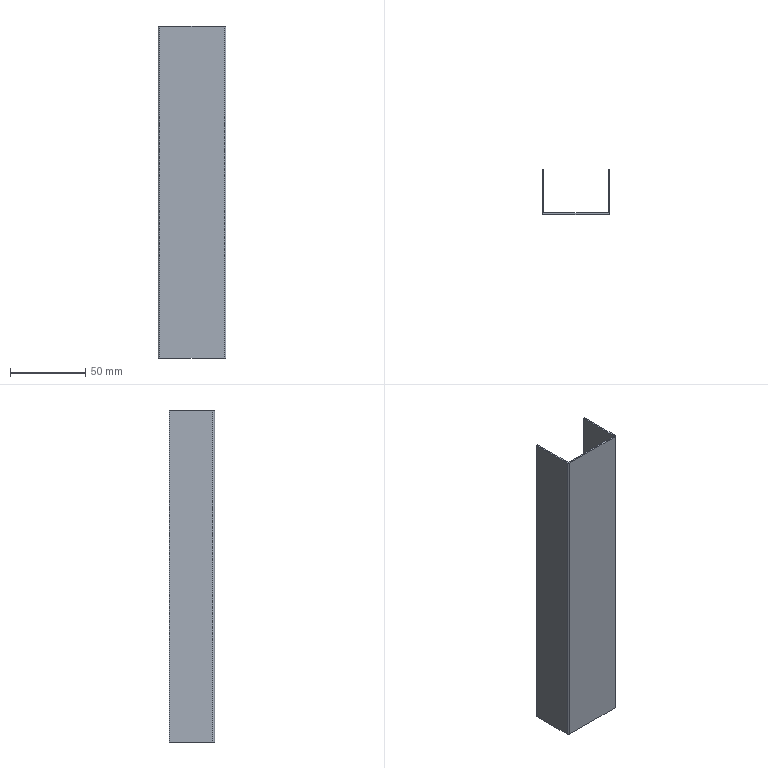Component | SolidWorks | WeldmentDrawing-1_WireDuct-1 | 1 solid | 22 faces | box 45 x 30 x 220 mm | volume 22547 mm3 | plane 18 | cylinder 4 | commonest cylinder face diameters 2.2 x2 0.2 x2
STEP:
#1=COLOUR_RGB('',0.7922,0.8196,0.9333);
#2=FILL_AREA_STYLE_COLOUR('',#1);
#3=FILL_AREA_STYLE('',(#2));
#4=SURFACE_STYLE_FILL_AREA(#3);
#5=SURFACE_SIDE_STYLE('',(#4));
#6=SURFACE_STYLE_USAGE(.BOTH.,#5);
#7=PRESENTATION_STYLE_ASSIGNMENT((#6));
#8=CARTESIAN_POINT('',(-6.554,2.411,-7.874));
#9=VERTEX_POINT('',#8);
#10=CARTESIAN_POINT('',(-8.239,2.411,-7.874));
#11=VERTEX_POINT('',#10);
#12=CARTESIAN_POINT('',(-8.282,2.411,-7.874));
#13=DIRECTION('',(-1.,0.,0.));
#14=VECTOR('',#13,39.37);
#15=LINE('',#12,#14);
#16=EDGE_CURVE('',#9,#11,#15,.T.);
#17=ORIENTED_EDGE('',*,*,#16,.F.);
#18=CARTESIAN_POINT('',(-6.554,2.411,0.7874));
#19=VERTEX_POINT('',#18);
#20=CARTESIAN_POINT('',(-6.554,2.411,-7.874));
#21=DIRECTION('',(0.,0.,1.));
#22=VECTOR('',#21,39.37);
#23=LINE('',#20,#22);
#24=EDGE_CURVE('',#9,#19,#23,.T.);
#25=ORIENTED_EDGE('',*,*,#24,.T.);
#26=CARTESIAN_POINT('',(-8.239,2.411,0.7874));
#27=VERTEX_POINT('',#26);
#28=CARTESIAN_POINT('',(-8.282,2.411,0.7874));
#29=DIRECTION('',(1.,0.,0.));
#30=VECTOR('',#29,39.37);
#31=LINE('',#28,#30);
#32=EDGE_CURVE('',#27,#19,#31,.T.);
#33=ORIENTED_EDGE('',*,*,#32,.F.);
#34=CARTESIAN_POINT('',(-8.239,2.411,0.7874));
#35=DIRECTION('',(0.,0.,-1.));
#36=VECTOR('',#35,39.37);
#37=LINE('',#34,#36);
#38=EDGE_CURVE('',#27,#11,#37,.T.);
#39=ORIENTED_EDGE('',*,*,#38,.T.);
#40=EDGE_LOOP('',(#17,#25,#33,#39));
#41=FACE_OUTER_BOUND('',#40,.T.);
#42=CARTESIAN_POINT('',(-6.765,2.411,-1.381));
#43=DIRECTION('',(0.,-1.,0.));
#44=DIRECTION('',(0.,0.,-1.));
#45=AXIS2_PLACEMENT_3D('',#42,#43,#44);
#46=PLANE('',#45);
#47=ADVANCED_FACE('',(#41),#46,.T.);
#48=CARTESIAN_POINT('',(-6.554,2.451,-7.874));
#49=VERTEX_POINT('',#48);
#50=CARTESIAN_POINT('',(-6.554,2.451,0.7874));
#51=VERTEX_POINT('',#50);
#52=CARTESIAN_POINT('',(-6.554,2.451,-7.874));
#53=DIRECTION('',(0.,0.,1.));
#54=VECTOR('',#53,39.37);
#55=LINE('',#52,#54);
#56=EDGE_CURVE('',#49,#51,#55,.T.);
#57=ORIENTED_EDGE('',*,*,#56,.F.);
#58=CARTESIAN_POINT('',(-8.239,2.451,-7.874));
#59=VERTEX_POINT('',#58);
#60=CARTESIAN_POINT('',(-8.282,2.451,-7.874));
#61=DIRECTION('',(-1.,0.,0.));
#62=VECTOR('',#61,39.37);
#63=LINE('',#60,#62);
#64=EDGE_CURVE('',#49,#59,#63,.T.);
#65=ORIENTED_EDGE('',*,*,#64,.T.);
#66=CARTESIAN_POINT('',(-8.239,2.451,0.7874));
#67=VERTEX_POINT('',#66);
#68=CARTESIAN_POINT('',(-8.239,2.451,0.7874));
#69=DIRECTION('',(0.,0.,-1.));
#70=VECTOR('',#69,39.37);
#71=LINE('',#68,#70);
#72=EDGE_CURVE('',#67,#59,#71,.T.);
#73=ORIENTED_EDGE('',*,*,#72,.F.);
#74=CARTESIAN_POINT('',(-8.282,2.451,0.7874));
#75=DIRECTION('',(1.,0.,0.));
#76=VECTOR('',#75,39.37);
#77=LINE('',#74,#76);
#78=EDGE_CURVE('',#67,#51,#77,.T.);
#79=ORIENTED_EDGE('',*,*,#78,.T.);
#80=EDGE_LOOP('',(#57,#65,#73,#79));
#81=FACE_OUTER_BOUND('',#80,.T.);
#82=CARTESIAN_POINT('',(-6.765,2.451,-1.381));
#83=DIRECTION('',(0.,-1.,0.));
#84=DIRECTION('',(0.,0.,-1.));
#85=AXIS2_PLACEMENT_3D('',#82,#83,#84);
#86=PLANE('',#85);
#87=ADVANCED_FACE('',(#81),#86,.F.);
#88=ORIENTED_EDGE('',*,*,#64,.F.);
#89=CARTESIAN_POINT('',(-6.554,2.451,-7.874));
#90=DIRECTION('',(0.,-1.,0.));
#91=VECTOR('',#90,39.37);
#92=LINE('',#89,#91);
#93=EDGE_CURVE('',#49,#9,#92,.T.);
#94=ORIENTED_EDGE('',*,*,#93,.T.);
#95=ORIENTED_EDGE('',*,*,#16,.T.);
#96=CARTESIAN_POINT('',(-8.239,2.451,-7.874));
#97=DIRECTION('',(0.,-1.,0.));
#98=VECTOR('',#97,39.37);
#99=LINE('',#96,#98);
#100=EDGE_CURVE('',#59,#11,#99,.T.);
#101=ORIENTED_EDGE('',*,*,#100,.F.);
#102=EDGE_LOOP('',(#88,#94,#95,#101));
#103=FACE_OUTER_BOUND('',#102,.T.);
#104=CARTESIAN_POINT('',(-8.282,2.411,-7.874));
#105=DIRECTION('',(0.,0.,-1.));
#106=DIRECTION('',(-1.,0.,0.));
#107=AXIS2_PLACEMENT_3D('',#104,#105,#106);
#108=PLANE('',#107);
#109=ADVANCED_FACE('',(#103),#108,.T.);
#110=CARTESIAN_POINT('',(-6.554,2.451,0.7874));
#111=DIRECTION('',(0.,-1.,0.));
#112=VECTOR('',#111,39.37);
#113=LINE('',#110,#112);
#114=EDGE_CURVE('',#51,#19,#113,.T.);
#115=ORIENTED_EDGE('',*,*,#114,.F.);
#116=ORIENTED_EDGE('',*,*,#78,.F.);
#117=CARTESIAN_POINT('',(-8.239,2.451,0.7874));
#118=DIRECTION('',(0.,-1.,0.));
#119=VECTOR('',#118,39.37);
#120=LINE('',#117,#119);
#121=EDGE_CURVE('',#67,#27,#120,.T.);
#122=ORIENTED_EDGE('',*,*,#121,.T.);
#123=ORIENTED_EDGE('',*,*,#32,.T.);
#124=EDGE_LOOP('',(#115,#116,#122,#123));
#125=FACE_OUTER_BOUND('',#124,.T.);
#126=CARTESIAN_POINT('',(-8.282,2.411,0.7874));
#127=DIRECTION('',(0.,0.,1.));
#128=DIRECTION('',(1.,0.,0.));
#129=AXIS2_PLACEMENT_3D('',#126,#127,#128);
#130=PLANE('',#129);
#131=ADVANCED_FACE('',(#125),#130,.T.);
#132=CARTESIAN_POINT('',(-8.243,2.455,-7.874));
#133=VERTEX_POINT('',#132);
#134=CARTESIAN_POINT('',(-8.282,2.455,-7.874));
#135=VERTEX_POINT('',#134);
#136=CARTESIAN_POINT('',(-8.282,2.455,-7.874));
#137=DIRECTION('',(-1.,-0.,0.));
#138=VECTOR('',#137,39.37);
#139=LINE('',#136,#138);
#140=EDGE_CURVE('',#133,#135,#139,.T.);
#141=ORIENTED_EDGE('',*,*,#140,.F.);
#142=CARTESIAN_POINT('',(-8.239,2.455,-7.874));
#143=DIRECTION('',(0.,0.,-1.));
#144=DIRECTION('',(1.,0.,0.));
#145=AXIS2_PLACEMENT_3D('',#142,#143,#144);
#146=CIRCLE('',#145,0.003937);
#147=EDGE_CURVE('',#59,#133,#146,.T.);
#148=ORIENTED_EDGE('',*,*,#147,.F.);
#149=ORIENTED_EDGE('',*,*,#100,.T.);
#150=CARTESIAN_POINT('',(-8.239,2.455,-7.874));
#151=DIRECTION('',(0.,0.,-1.));
#152=DIRECTION('',(1.,0.,0.));
#153=AXIS2_PLACEMENT_3D('',#150,#151,#152);
#154=CIRCLE('',#153,0.04331);
#155=EDGE_CURVE('',#11,#135,#154,.T.);
#156=ORIENTED_EDGE('',*,*,#155,.T.);
#157=EDGE_LOOP('',(#141,#148,#149,#156));
#158=FACE_OUTER_BOUND('',#157,.T.);
#159=CARTESIAN_POINT('',(-8.239,2.455,-7.874));
#160=DIRECTION('',(0.,0.,-1.));
#161=DIRECTION('',(-1.,0.,0.));
#162=AXIS2_PLACEMENT_3D('',#159,#160,#161);
#163=PLANE('',#162);
#164=ADVANCED_FACE('',(#158),#163,.T.);
#165=CARTESIAN_POINT('',(-8.243,2.455,0.7874));
#166=VERTEX_POINT('',#165);
#167=CARTESIAN_POINT('',(-8.239,2.455,0.7874));
#168=DIRECTION('',(0.,0.,1.));
#169=DIRECTION('',(1.,0.,0.));
#170=AXIS2_PLACEMENT_3D('',#167,#168,#169);
#171=CIRCLE('',#170,0.003937);
#172=EDGE_CURVE('',#166,#67,#171,.T.);
#173=ORIENTED_EDGE('',*,*,#172,.F.);
#174=CARTESIAN_POINT('',(-8.282,2.455,0.7874));
#175=VERTEX_POINT('',#174);
#176=CARTESIAN_POINT('',(-8.243,2.455,0.7874));
#177=DIRECTION('',(-1.,-0.,0.));
#178=VECTOR('',#177,39.37);
#179=LINE('',#176,#178);
#180=EDGE_CURVE('',#166,#175,#179,.T.);
#181=ORIENTED_EDGE('',*,*,#180,.T.);
#182=CARTESIAN_POINT('',(-8.239,2.455,0.7874));
#183=DIRECTION('',(0.,0.,1.));
#184=DIRECTION('',(1.,0.,0.));
#185=AXIS2_PLACEMENT_3D('',#182,#183,#184);
#186=CIRCLE('',#185,0.04331);
#187=EDGE_CURVE('',#175,#27,#186,.T.);
#188=ORIENTED_EDGE('',*,*,#187,.T.);
#189=ORIENTED_EDGE('',*,*,#121,.F.);
#190=EDGE_LOOP('',(#173,#181,#188,#189));
#191=FACE_OUTER_BOUND('',#190,.T.);
#192=CARTESIAN_POINT('',(-8.239,2.455,0.7874));
#193=DIRECTION('',(0.,0.,-1.));
#194=DIRECTION('',(-1.,0.,0.));
#195=AXIS2_PLACEMENT_3D('',#192,#193,#194);
#196=PLANE('',#195);
#197=ADVANCED_FACE('',(#191),#196,.F.);
#198=ORIENTED_EDGE('',*,*,#38,.F.);
#199=ORIENTED_EDGE('',*,*,#187,.F.);
#200=CARTESIAN_POINT('',(-8.282,2.455,-7.874));
#201=DIRECTION('',(0.,0.,-1.));
#202=VECTOR('',#201,39.37);
#203=LINE('',#200,#202);
#204=EDGE_CURVE('',#175,#135,#203,.T.);
#205=ORIENTED_EDGE('',*,*,#204,.T.);
#206=ORIENTED_EDGE('',*,*,#155,.F.);
#207=EDGE_LOOP('',(#198,#199,#205,#206));
#208=FACE_OUTER_BOUND('',#207,.T.);
#209=CARTESIAN_POINT('',(-8.239,2.455,0.7874));
#210=DIRECTION('',(0.,0.,1.));
#211=DIRECTION('',(-1.,-0.,0.));
#212=AXIS2_PLACEMENT_3D('',#209,#210,#211);
#213=CYLINDRICAL_SURFACE('',#212,0.04331);
#214=ADVANCED_FACE('',(#208),#213,.T.);
#215=ORIENTED_EDGE('',*,*,#72,.T.);
#216=ORIENTED_EDGE('',*,*,#147,.T.);
#217=CARTESIAN_POINT('',(-8.243,2.455,-7.874));
#218=DIRECTION('',(0.,0.,1.));
#219=VECTOR('',#218,39.37);
#220=LINE('',#217,#219);
#221=EDGE_CURVE('',#133,#166,#220,.T.);
#222=ORIENTED_EDGE('',*,*,#221,.T.);
#223=ORIENTED_EDGE('',*,*,#172,.T.);
#224=EDGE_LOOP('',(#215,#216,#222,#223));
#225=FACE_OUTER_BOUND('',#224,.T.);
#226=CARTESIAN_POINT('',(-8.239,2.455,0.7874));
#227=DIRECTION('',(0.,0.,1.));
#228=DIRECTION('',(-1.,0.,0.));
#229=AXIS2_PLACEMENT_3D('',#226,#227,#228);
#230=CYLINDRICAL_SURFACE('',#229,0.003937);
#231=ADVANCED_FACE('',(#225),#230,.F.);
#232=ORIENTED_EDGE('',*,*,#180,.F.);
#233=CARTESIAN_POINT('',(-8.243,3.592,0.7874));
#234=VERTEX_POINT('',#233);
#235=CARTESIAN_POINT('',(-8.243,3.592,0.7874));
#236=DIRECTION('',(-0.,1.,0.));
#237=VECTOR('',#236,39.37);
#238=LINE('',#235,#237);
#239=EDGE_CURVE('',#166,#234,#238,.T.);
#240=ORIENTED_EDGE('',*,*,#239,.T.);
#241=CARTESIAN_POINT('',(-8.282,3.592,0.7874));
#242=VERTEX_POINT('',#241);
#243=CARTESIAN_POINT('',(-8.282,3.592,0.7874));
#244=DIRECTION('',(1.,0.,0.));
#245=VECTOR('',#244,39.37);
#246=LINE('',#243,#245);
#247=EDGE_CURVE('',#242,#234,#246,.T.);
#248=ORIENTED_EDGE('',*,*,#247,.F.);
#249=CARTESIAN_POINT('',(-8.282,2.451,0.7874));
#250=DIRECTION('',(-0.,1.,0.));
#251=VECTOR('',#250,39.37);
#252=LINE('',#249,#251);
#253=EDGE_CURVE('',#175,#242,#252,.T.);
#254=ORIENTED_EDGE('',*,*,#253,.F.);
#255=EDGE_LOOP('',(#232,#240,#248,#254));
#256=FACE_OUTER_BOUND('',#255,.T.);
#257=CARTESIAN_POINT('',(-8.282,3.592,0.7874));
#258=DIRECTION('',(0.,0.,-1.));
#259=DIRECTION('',(-1.,0.,0.));
#260=AXIS2_PLACEMENT_3D('',#257,#258,#259);
#261=PLANE('',#260);
#262=ADVANCED_FACE('',(#256),#261,.F.);
#263=ORIENTED_EDGE('',*,*,#140,.T.);
#264=CARTESIAN_POINT('',(-8.282,3.592,-7.874));
#265=VERTEX_POINT('',#264);
#266=CARTESIAN_POINT('',(-8.282,2.451,-7.874));
#267=DIRECTION('',(0.,-1.,0.));
#268=VECTOR('',#267,39.37);
#269=LINE('',#266,#268);
#270=EDGE_CURVE('',#265,#135,#269,.T.);
#271=ORIENTED_EDGE('',*,*,#270,.F.);
#272=CARTESIAN_POINT('',(-8.243,3.592,-7.874));
#273=VERTEX_POINT('',#272);
#274=CARTESIAN_POINT('',(-8.282,3.592,-7.874));
#275=DIRECTION('',(1.,0.,0.));
#276=VECTOR('',#275,39.37);
#277=LINE('',#274,#276);
#278=EDGE_CURVE('',#265,#273,#277,.T.);
#279=ORIENTED_EDGE('',*,*,#278,.T.);
#280=CARTESIAN_POINT('',(-8.243,2.451,-7.874));
#281=DIRECTION('',(0.,-1.,0.));
#282=VECTOR('',#281,39.37);
#283=LINE('',#280,#282);
#284=EDGE_CURVE('',#273,#133,#283,.T.);
#285=ORIENTED_EDGE('',*,*,#284,.T.);
#286=EDGE_LOOP('',(#263,#271,#279,#285));
#287=FACE_OUTER_BOUND('',#286,.T.);
#288=CARTESIAN_POINT('',(-8.282,2.451,-7.874));
#289=DIRECTION('',(0.,0.,1.));
#290=DIRECTION('',(1.,0.,0.));
#291=AXIS2_PLACEMENT_3D('',#288,#289,#290);
#292=PLANE('',#291);
#293=ADVANCED_FACE('',(#287),#292,.F.);
#294=ORIENTED_EDGE('',*,*,#204,.F.);
#295=ORIENTED_EDGE('',*,*,#253,.T.);
#296=CARTESIAN_POINT('',(-8.282,3.592,-1.381));
#297=DIRECTION('',(0.,0.,-1.));
#298=VECTOR('',#297,39.37);
#299=LINE('',#296,#298);
#300=EDGE_CURVE('',#242,#265,#299,.T.);
#301=ORIENTED_EDGE('',*,*,#300,.T.);
#302=ORIENTED_EDGE('',*,*,#270,.T.);
#303=EDGE_LOOP('',(#294,#295,#301,#302));
#304=FACE_OUTER_BOUND('',#303,.T.);
#305=CARTESIAN_POINT('',(-8.282,2.451,-1.381));
#306=DIRECTION('',(1.,0.,0.));
#307=DIRECTION('',(-0.,1.,0.));
#308=AXIS2_PLACEMENT_3D('',#305,#306,#307);
#309=PLANE('',#308);
#310=ADVANCED_FACE('',(#304),#309,.F.);
#311=ORIENTED_EDGE('',*,*,#239,.F.);
#312=ORIENTED_EDGE('',*,*,#221,.F.);
#313=ORIENTED_EDGE('',*,*,#284,.F.);
#314=CARTESIAN_POINT('',(-8.243,3.592,-7.874));
#315=DIRECTION('',(0.,0.,-1.));
#316=VECTOR('',#315,39.37);
#317=LINE('',#314,#316);
#318=EDGE_CURVE('',#234,#273,#317,.T.);
#319=ORIENTED_EDGE('',*,*,#318,.F.);
#320=EDGE_LOOP('',(#311,#312,#313,#319));
#321=FACE_OUTER_BOUND('',#320,.T.);
#322=CARTESIAN_POINT('',(-8.243,2.451,-1.381));
#323=DIRECTION('',(1.,0.,0.));
#324=DIRECTION('',(-0.,1.,0.));
#325=AXIS2_PLACEMENT_3D('',#322,#323,#324);
#326=PLANE('',#325);
#327=ADVANCED_FACE('',(#321),#326,.T.);
#328=ORIENTED_EDGE('',*,*,#318,.T.);
#329=ORIENTED_EDGE('',*,*,#278,.F.);
#330=ORIENTED_EDGE('',*,*,#300,.F.);
#331=ORIENTED_EDGE('',*,*,#247,.T.);
#332=EDGE_LOOP('',(#328,#329,#330,#331));
#333=FACE_OUTER_BOUND('',#332,.T.);
#334=CARTESIAN_POINT('',(-8.282,3.592,-7.874));
#335=DIRECTION('',(0.,-1.,0.));
#336=DIRECTION('',(1.,0.,0.));
#337=AXIS2_PLACEMENT_3D('',#334,#335,#336);
#338=PLANE('',#337);
#339=ADVANCED_FACE('',(#333),#338,.F.);
#340=CARTESIAN_POINT('',(-6.55,2.455,0.7874));
#341=VERTEX_POINT('',#340);
#342=CARTESIAN_POINT('',(-6.51,2.455,0.7874));
#343=VERTEX_POINT('',#342);
#344=CARTESIAN_POINT('',(-6.51,2.455,0.7874));
#345=DIRECTION('',(1.,-0.,0.));
#346=VECTOR('',#345,39.37);
#347=LINE('',#344,#346);
#348=EDGE_CURVE('',#341,#343,#347,.T.);
#349=ORIENTED_EDGE('',*,*,#348,.F.);
#350=CARTESIAN_POINT('',(-6.554,2.455,0.7874));
#351=DIRECTION('',(0.,0.,1.));
#352=DIRECTION('',(-1.,0.,0.));
#353=AXIS2_PLACEMENT_3D('',#350,#351,#352);
#354=CIRCLE('',#353,0.003937);
#355=EDGE_CURVE('',#51,#341,#354,.T.);
#356=ORIENTED_EDGE('',*,*,#355,.F.);
#357=ORIENTED_EDGE('',*,*,#114,.T.);
#358=CARTESIAN_POINT('',(-6.554,2.455,0.7874));
#359=DIRECTION('',(0.,0.,1.));
#360=DIRECTION('',(-1.,0.,0.));
#361=AXIS2_PLACEMENT_3D('',#358,#359,#360);
#362=CIRCLE('',#361,0.04331);
#363=EDGE_CURVE('',#19,#343,#362,.T.);
#364=ORIENTED_EDGE('',*,*,#363,.T.);
#365=EDGE_LOOP('',(#349,#356,#357,#364));
#366=FACE_OUTER_BOUND('',#365,.T.);
#367=CARTESIAN_POINT('',(-6.554,2.455,0.7874));
#368=DIRECTION('',(0.,0.,1.));
#369=DIRECTION('',(1.,0.,0.));
#370=AXIS2_PLACEMENT_3D('',#367,#368,#369);
#371=PLANE('',#370);
#372=ADVANCED_FACE('',(#366),#371,.T.);
#373=CARTESIAN_POINT('',(-6.55,2.455,-7.874));
#374=VERTEX_POINT('',#373);
#375=CARTESIAN_POINT('',(-6.554,2.455,-7.874));
#376=DIRECTION('',(0.,0.,-1.));
#377=DIRECTION('',(-1.,0.,0.));
#378=AXIS2_PLACEMENT_3D('',#375,#376,#377);
#379=CIRCLE('',#378,0.003937);
#380=EDGE_CURVE('',#374,#49,#379,.T.);
#381=ORIENTED_EDGE('',*,*,#380,.F.);
#382=CARTESIAN_POINT('',(-6.51,2.455,-7.874));
#383=VERTEX_POINT('',#382);
#384=CARTESIAN_POINT('',(-6.55,2.455,-7.874));
#385=DIRECTION('',(1.,-0.,0.));
#386=VECTOR('',#385,39.37);
#387=LINE('',#384,#386);
#388=EDGE_CURVE('',#374,#383,#387,.T.);
#389=ORIENTED_EDGE('',*,*,#388,.T.);
#390=CARTESIAN_POINT('',(-6.554,2.455,-7.874));
#391=DIRECTION('',(0.,0.,-1.));
#392=DIRECTION('',(-1.,0.,0.));
#393=AXIS2_PLACEMENT_3D('',#390,#391,#392);
#394=CIRCLE('',#393,0.04331);
#395=EDGE_CURVE('',#383,#9,#394,.T.);
#396=ORIENTED_EDGE('',*,*,#395,.T.);
#397=ORIENTED_EDGE('',*,*,#93,.F.);
#398=EDGE_LOOP('',(#381,#389,#396,#397));
#399=FACE_OUTER_BOUND('',#398,.T.);
#400=CARTESIAN_POINT('',(-6.554,2.455,-7.874));
#401=DIRECTION('',(0.,0.,1.));
#402=DIRECTION('',(1.,0.,0.));
#403=AXIS2_PLACEMENT_3D('',#400,#401,#402);
#404=PLANE('',#403);
#405=ADVANCED_FACE('',(#399),#404,.F.);
#406=ORIENTED_EDGE('',*,*,#24,.F.);
#407=ORIENTED_EDGE('',*,*,#395,.F.);
#408=CARTESIAN_POINT('',(-6.51,2.455,0.7874));
#409=DIRECTION('',(-0.,-0.,1.));
#410=VECTOR('',#409,39.37);
#411=LINE('',#408,#410);
#412=EDGE_CURVE('',#383,#343,#411,.T.);
#413=ORIENTED_EDGE('',*,*,#412,.T.);
#414=ORIENTED_EDGE('',*,*,#363,.F.);
#415=EDGE_LOOP('',(#406,#407,#413,#414));
#416=FACE_OUTER_BOUND('',#415,.T.);
#417=CARTESIAN_POINT('',(-6.554,2.455,-7.874));
#418=DIRECTION('',(0.,0.,-1.));
#419=DIRECTION('',(1.,-0.,0.));
#420=AXIS2_PLACEMENT_3D('',#417,#418,#419);
#421=CYLINDRICAL_SURFACE('',#420,0.04331);
#422=ADVANCED_FACE('',(#416),#421,.T.);
#423=ORIENTED_EDGE('',*,*,#56,.T.);
#424=ORIENTED_EDGE('',*,*,#355,.T.);
#425=CARTESIAN_POINT('',(-6.55,2.455,0.7874));
#426=DIRECTION('',(0.,0.,-1.));
#427=VECTOR('',#426,39.37);
#428=LINE('',#425,#427);
#429=EDGE_CURVE('',#341,#374,#428,.T.);
#430=ORIENTED_EDGE('',*,*,#429,.T.);
#431=ORIENTED_EDGE('',*,*,#380,.T.);
#432=EDGE_LOOP('',(#423,#424,#430,#431));
#433=FACE_OUTER_BOUND('',#432,.T.);
#434=CARTESIAN_POINT('',(-6.554,2.455,-7.874));
#435=DIRECTION('',(0.,0.,-1.));
#436=DIRECTION('',(1.,0.,0.));
#437=AXIS2_PLACEMENT_3D('',#434,#435,#436);
#438=CYLINDRICAL_SURFACE('',#437,0.003937);
#439=ADVANCED_FACE('',(#433),#438,.F.);
#440=ORIENTED_EDGE('',*,*,#348,.T.);
#441=CARTESIAN_POINT('',(-6.51,3.592,0.7874));
#442=VERTEX_POINT('',#441);
#443=CARTESIAN_POINT('',(-6.51,2.451,0.7874));
#444=DIRECTION('',(-0.,-1.,0.));
#445=VECTOR('',#444,39.37);
#446=LINE('',#443,#445);
#447=EDGE_CURVE('',#442,#343,#446,.T.);
#448=ORIENTED_EDGE('',*,*,#447,.F.);
#449=CARTESIAN_POINT('',(-6.55,3.592,0.7874));
#450=VERTEX_POINT('',#449);
#451=CARTESIAN_POINT('',(-6.51,3.592,0.7874));
#452=DIRECTION('',(-1.,0.,0.));
#453=VECTOR('',#452,39.37);
#454=LINE('',#451,#453);
#455=EDGE_CURVE('',#442,#450,#454,.T.);
#456=ORIENTED_EDGE('',*,*,#455,.T.);
#457=CARTESIAN_POINT('',(-6.55,2.451,0.7874));
#458=DIRECTION('',(-0.,-1.,0.));
#459=VECTOR('',#458,39.37);
#460=LINE('',#457,#459);
#461=EDGE_CURVE('',#450,#341,#460,.T.);
#462=ORIENTED_EDGE('',*,*,#461,.T.);
#463=EDGE_LOOP('',(#440,#448,#456,#462));
#464=FACE_OUTER_BOUND('',#463,.T.);
#465=CARTESIAN_POINT('',(-6.51,2.451,0.7874));
#466=DIRECTION('',(0.,0.,-1.));
#467=DIRECTION('',(-1.,0.,0.));
#468=AXIS2_PLACEMENT_3D('',#465,#466,#467);
#469=PLANE('',#468);
#470=ADVANCED_FACE('',(#464),#469,.F.);
#471=ORIENTED_EDGE('',*,*,#388,.F.);
#472=CARTESIAN_POINT('',(-6.55,3.592,-7.874));
#473=VERTEX_POINT('',#472);
#474=CARTESIAN_POINT('',(-6.55,3.592,-7.874));
#475=DIRECTION('',(0.,1.,0.));
#476=VECTOR('',#475,39.37);
#477=LINE('',#474,#476);
#478=EDGE_CURVE('',#374,#473,#477,.T.);
#479=ORIENTED_EDGE('',*,*,#478,.T.);
#480=CARTESIAN_POINT('',(-6.51,3.592,-7.874));
#481=VERTEX_POINT('',#480);
#482=CARTESIAN_POINT('',(-6.51,3.592,-7.874));
#483=DIRECTION('',(-1.,0.,0.));
#484=VECTOR('',#483,39.37);
#485=LINE('',#482,#484);
#486=EDGE_CURVE('',#481,#473,#485,.T.);
#487=ORIENTED_EDGE('',*,*,#486,.F.);
#488=CARTESIAN_POINT('',(-6.51,2.451,-7.874));
#489=DIRECTION('',(0.,1.,0.));
#490=VECTOR('',#489,39.37);
#491=LINE('',#488,#490);
#492=EDGE_CURVE('',#383,#481,#491,.T.);
#493=ORIENTED_EDGE('',*,*,#492,.F.);
#494=EDGE_LOOP('',(#471,#479,#487,#493));
#495=FACE_OUTER_BOUND('',#494,.T.);
#496=CARTESIAN_POINT('',(-6.51,3.592,-7.874));
#497=DIRECTION('',(0.,0.,1.));
#498=DIRECTION('',(1.,0.,0.));
#499=AXIS2_PLACEMENT_3D('',#496,#497,#498);
#500=PLANE('',#499);
#501=ADVANCED_FACE('',(#495),#500,.F.);
#502=ORIENTED_EDGE('',*,*,#412,.F.);
#503=ORIENTED_EDGE('',*,*,#492,.T.);
#504=CARTESIAN_POINT('',(-6.51,3.592,-1.381));
#505=DIRECTION('',(0.,0.,1.));
#506=VECTOR('',#505,39.37);
#507=LINE('',#504,#506);
#508=EDGE_CURVE('',#481,#442,#507,.T.);
#509=ORIENTED_EDGE('',*,*,#508,.T.);
#510=ORIENTED_EDGE('',*,*,#447,.T.);
#511=EDGE_LOOP('',(#502,#503,#509,#510));
#512=FACE_OUTER_BOUND('',#511,.T.);
#513=CARTESIAN_POINT('',(-6.51,2.451,-1.381));
#514=DIRECTION('',(-1.,0.,0.));
#515=DIRECTION('',(-0.,-1.,0.));
#516=AXIS2_PLACEMENT_3D('',#513,#514,#515);
#517=PLANE('',#516);
#518=ADVANCED_FACE('',(#512),#517,.F.);
#519=ORIENTED_EDGE('',*,*,#478,.F.);
#520=ORIENTED_EDGE('',*,*,#429,.F.);
#521=ORIENTED_EDGE('',*,*,#461,.F.);
#522=CARTESIAN_POINT('',(-6.55,3.592,0.7874));
#523=DIRECTION('',(0.,0.,1.));
#524=VECTOR('',#523,39.37);
#525=LINE('',#522,#524);
#526=EDGE_CURVE('',#473,#450,#525,.T.);
#527=ORIENTED_EDGE('',*,*,#526,.F.);
#528=EDGE_LOOP('',(#519,#520,#521,#527));
#529=FACE_OUTER_BOUND('',#528,.T.);
#530=CARTESIAN_POINT('',(-6.55,2.451,-1.381));
#531=DIRECTION('',(-1.,0.,0.));
#532=DIRECTION('',(-0.,-1.,0.));
#533=AXIS2_PLACEMENT_3D('',#530,#531,#532);
#534=PLANE('',#533);
#535=ADVANCED_FACE('',(#529),#534,.T.);
#536=ORIENTED_EDGE('',*,*,#526,.T.);
#537=ORIENTED_EDGE('',*,*,#455,.F.);
#538=ORIENTED_EDGE('',*,*,#508,.F.);
#539=ORIENTED_EDGE('',*,*,#486,.T.);
#540=EDGE_LOOP('',(#536,#537,#538,#539));
#541=FACE_OUTER_BOUND('',#540,.T.);
#542=CARTESIAN_POINT('',(-6.51,3.592,0.7874));
#543=DIRECTION('',(-0.,-1.,0.));
#544=DIRECTION('',(1.,-0.,0.));
#545=AXIS2_PLACEMENT_3D('',#542,#543,#544);
#546=PLANE('',#545);
#547=ADVANCED_FACE('',(#541),#546,.F.);
#548=CLOSED_SHELL('',(#47,#87,#109,#131,#164,#197,#214,#231,#262,#293,#310,#327,#339,#372,#405,#422,#439,#470,#501,#518,#535,#547));
#549=MANIFOLD_SOLID_BREP('',#548);
#550=STYLED_ITEM('',(#7),#549);
#551=PRESENTATION_LAYER_ASSIGNMENT('','',(#550));
#552=(LENGTH_UNIT()NAMED_UNIT(*)SI_UNIT($,.METRE.));
#553=LENGTH_MEASURE_WITH_UNIT(LENGTH_MEASURE(0.0254),#552);
#554=DIMENSIONAL_EXPONENTS(1.,0.,0.,0.,0.,0.,0.);
#555=(CONVERSION_BASED_UNIT('',#553)LENGTH_UNIT()NAMED_UNIT(#554));
#556=UNCERTAINTY_MEASURE_WITH_UNIT(LENGTH_MEASURE(0.00001),#555,'','');
#557=(NAMED_UNIT(*)PLANE_ANGLE_UNIT()SI_UNIT($,.RADIAN.));
#558=(NAMED_UNIT(*)SI_UNIT($,.STERADIAN.)SOLID_ANGLE_UNIT());
#559=(GEOMETRIC_REPRESENTATION_CONTEXT(3)GLOBAL_UNCERTAINTY_ASSIGNED_CONTEXT((#556))GLOBAL_UNIT_ASSIGNED_CONTEXT((#555,#557,#558))REPRESENTATION_CONTEXT('',''));
#560=MECHANICAL_DESIGN_GEOMETRIC_PRESENTATION_REPRESENTATION('',(#550),#559);
#561=CARTESIAN_POINT('',(0.,0.,0.));
#562=DIRECTION('',(0.,0.,1.));
#563=DIRECTION('',(1.,0.,0.));
#564=AXIS2_PLACEMENT_3D('',#561,#562,#563);
#565=(LENGTH_UNIT()NAMED_UNIT(*)SI_UNIT($,.METRE.));
#566=LENGTH_MEASURE_WITH_UNIT(LENGTH_MEASURE(0.0254),#565);
#567=DIMENSIONAL_EXPONENTS(1.,0.,0.,0.,0.,0.,0.);
#568=(CONVERSION_BASED_UNIT('',#566)LENGTH_UNIT()NAMED_UNIT(#567));
#569=UNCERTAINTY_MEASURE_WITH_UNIT(LENGTH_MEASURE(0.00001),#568,'','');
#570=(NAMED_UNIT(*)PLANE_ANGLE_UNIT()SI_UNIT($,.RADIAN.));
#571=(NAMED_UNIT(*)SI_UNIT($,.STERADIAN.)SOLID_ANGLE_UNIT());
#572=(GEOMETRIC_REPRESENTATION_CONTEXT(3)GLOBAL_UNCERTAINTY_ASSIGNED_CONTEXT((#569))GLOBAL_UNIT_ASSIGNED_CONTEXT((#568,#570,#571))REPRESENTATION_CONTEXT('',''));
#573=ADVANCED_BREP_SHAPE_REPRESENTATION('',(#549,#564),#572);